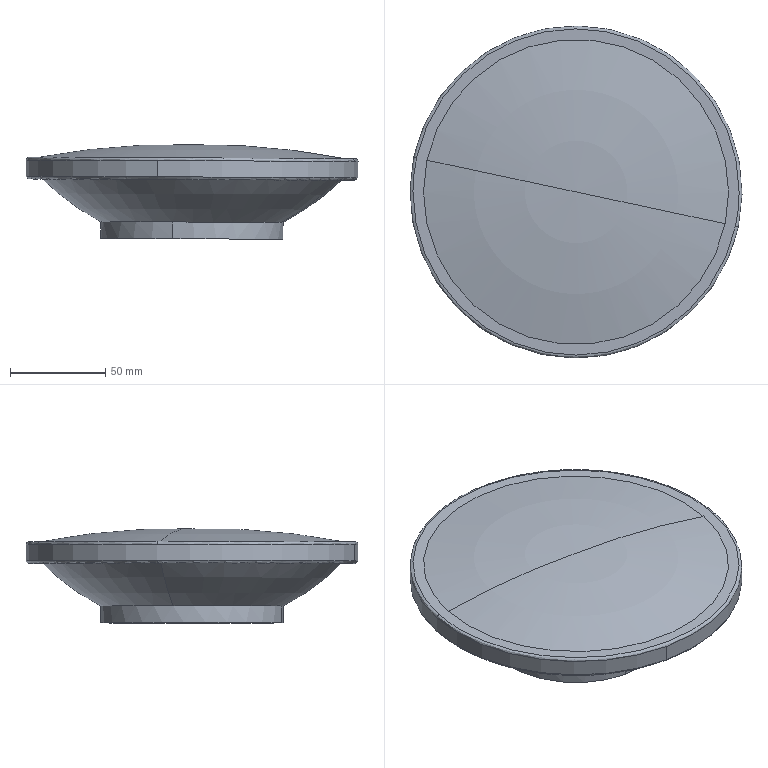Component | SolidWorks | Light-1_GreenLight-1 | 1 solid | 15 faces | box 174.03 x 174 x 49.62 mm | volume 703261 mm3 | cylinder 4 | torus 4 | spline 4 | plane 3 | commonest cylinder face diameters 95.736 x2 174 x2
STEP:
#1=COLOUR_RGB('',0.7922,0.8196,0.9333);
#2=FILL_AREA_STYLE_COLOUR('',#1);
#3=FILL_AREA_STYLE('',(#2));
#4=SURFACE_STYLE_FILL_AREA(#3);
#5=SURFACE_SIDE_STYLE('',(#4));
#6=SURFACE_STYLE_USAGE(.BOTH.,#5);
#7=PRESENTATION_STYLE_ASSIGNMENT((#6));
#8=CARTESIAN_POINT('',(-212.,267.71,12.424));
#9=VERTEX_POINT('',#8);
#10=CARTESIAN_POINT('',(-212.786,264.024,12.427));
#11=VERTEX_POINT('',#10);
#12=CARTESIAN_POINT('',(-212.393,265.867,12.425));
#13=DIRECTION('',(-0.004294,-0.,-1.));
#14=DIRECTION('',(-0.2083,-0.9781,0.0008945));
#15=AXIS2_PLACEMENT_3D('',#12,#13,#14);
#16=CIRCLE('',#15,1.885);
#17=EDGE_CURVE('',#9,#11,#16,.T.);
#18=ORIENTED_EDGE('',*,*,#17,.F.);
#19=CARTESIAN_POINT('',(-211.999,267.71,12.771));
#20=VERTEX_POINT('',#19);
#21=CARTESIAN_POINT('',(-212.,267.71,12.424));
#22=DIRECTION('',(0.004294,0.,1.));
#23=VECTOR('',#22,39.37);
#24=LINE('',#21,#23);
#25=EDGE_CURVE('',#9,#20,#24,.T.);
#26=ORIENTED_EDGE('',*,*,#25,.T.);
#27=CARTESIAN_POINT('',(-210.548,265.474,12.764));
#28=VERTEX_POINT('',#27);
#29=CARTESIAN_POINT('',(-212.392,265.867,12.772));
#30=DIRECTION('',(0.004294,0.,1.));
#31=DIRECTION('',(-0.978,0.2083,0.004199));
#32=AXIS2_PLACEMENT_3D('',#29,#30,#31);
#33=CIRCLE('',#32,1.885);
#34=EDGE_CURVE('',#28,#20,#33,.T.);
#35=ORIENTED_EDGE('',*,*,#34,.F.);
#36=CARTESIAN_POINT('',(-212.784,264.024,12.774));
#37=VERTEX_POINT('',#36);
#38=CARTESIAN_POINT('',(-212.392,265.867,12.772));
#39=DIRECTION('',(0.004294,0.,1.));
#40=DIRECTION('',(-0.978,0.2083,0.004199));
#41=AXIS2_PLACEMENT_3D('',#38,#39,#40);
#42=CIRCLE('',#41,1.885);
#43=EDGE_CURVE('',#37,#28,#42,.T.);
#44=ORIENTED_EDGE('',*,*,#43,.F.);
#45=CARTESIAN_POINT('',(-212.786,264.024,12.427));
#46=DIRECTION('',(0.004294,0.,1.));
#47=VECTOR('',#46,39.37);
#48=LINE('',#45,#47);
#49=EDGE_CURVE('',#11,#37,#48,.T.);
#50=ORIENTED_EDGE('',*,*,#49,.F.);
#51=EDGE_LOOP('',(#18,#26,#35,#44,#50));
#52=FACE_OUTER_BOUND('',#51,.T.);
#53=CARTESIAN_POINT('',(-212.393,265.867,12.425));
#54=DIRECTION('',(0.004294,0.,1.));
#55=DIRECTION('',(-0.2083,-0.9781,0.0008945));
#56=AXIS2_PLACEMENT_3D('',#53,#54,#55);
#57=CYLINDRICAL_SURFACE('',#56,1.885);
#58=ADVANCED_FACE('',(#52),#57,.T.);
#59=CARTESIAN_POINT('',(-214.235,266.26,12.78));
#60=VERTEX_POINT('',#59);
#61=CARTESIAN_POINT('',(-212.392,265.867,12.772));
#62=DIRECTION('',(0.004294,0.,1.));
#63=DIRECTION('',(-0.978,0.2083,0.004199));
#64=AXIS2_PLACEMENT_3D('',#61,#62,#63);
#65=CIRCLE('',#64,1.885);
#66=EDGE_CURVE('',#60,#37,#65,.T.);
#67=ORIENTED_EDGE('',*,*,#66,.T.);
#68=ORIENTED_EDGE('',*,*,#43,.T.);
#69=CARTESIAN_POINT('',(-209.309,265.211,13.689));
#70=VERTEX_POINT('',#69);
#71=CARTESIAN_POINT('',(-212.93,265.986,17.433));
#72=DIRECTION('',(-0.2083,-0.9781,0.0008945));
#73=DIRECTION('',(0.9781,-0.2083,0.));
#74=AXIS2_PLACEMENT_3D('',#71,#72,#73);
#75=CIRCLE('',#74,5.266);
#76=EDGE_CURVE('',#28,#70,#75,.T.);
#77=ORIENTED_EDGE('',*,*,#76,.T.);
#78=CARTESIAN_POINT('',(-215.466,266.523,13.716));
#79=VERTEX_POINT('',#78);
#80=CARTESIAN_POINT('',(-212.388,265.867,13.702));
#81=DIRECTION('',(-0.004294,-0.,-1.));
#82=DIRECTION('',(-0.978,0.2083,0.004199));
#83=AXIS2_PLACEMENT_3D('',#80,#81,#82);
#84=CIRCLE('',#83,3.148);
#85=EDGE_CURVE('',#70,#79,#84,.T.);
#86=ORIENTED_EDGE('',*,*,#85,.T.);
#87=CARTESIAN_POINT('',(-211.813,265.748,17.428));
#88=DIRECTION('',(0.2083,0.9781,-0.0008945));
#89=DIRECTION('',(-0.9781,0.2083,0.));
#90=AXIS2_PLACEMENT_3D('',#87,#88,#89);
#91=CIRCLE('',#90,5.266);
#92=EDGE_CURVE('',#60,#79,#91,.T.);
#93=ORIENTED_EDGE('',*,*,#92,.F.);
#94=EDGE_LOOP('',(#67,#68,#77,#86,#93));
#95=FACE_OUTER_BOUND('',#94,.T.);
#96=CARTESIAN_POINT('',(-212.372,265.867,17.431));
#97=DIRECTION('',(0.004294,0.,1.));
#98=DIRECTION('',(-0.978,0.2083,0.004199));
#99=AXIS2_PLACEMENT_3D('',#96,#97,#98);
#100=TOROIDAL_SURFACE('',#99,-0.5709,5.266);
#101=ADVANCED_FACE('',(#95),#100,.T.);
#102=CARTESIAN_POINT('',(-211.674,269.217,13.699));
#103=VERTEX_POINT('',#102);
#104=CARTESIAN_POINT('',(-209.038,265.154,13.688));
#105=VERTEX_POINT('',#104);
#106=CARTESIAN_POINT('',(-212.388,265.867,13.702));
#107=DIRECTION('',(-0.004294,-0.,-1.));
#108=DIRECTION('',(0.978,-0.2083,-0.004199));
#109=AXIS2_PLACEMENT_3D('',#106,#107,#108);
#110=CIRCLE('',#109,3.425);
#111=EDGE_CURVE('',#103,#105,#110,.T.);
#112=ORIENTED_EDGE('',*,*,#111,.F.);
#113=CARTESIAN_POINT('',(-211.673,269.217,14.034));
#114=VERTEX_POINT('',#113);
#115=CARTESIAN_POINT('',(-211.674,269.217,13.699));
#116=DIRECTION('',(0.004294,0.,1.));
#117=VECTOR('',#116,39.37);
#118=LINE('',#115,#117);
#119=EDGE_CURVE('',#103,#114,#118,.T.);
#120=ORIENTED_EDGE('',*,*,#119,.T.);
#121=CARTESIAN_POINT('',(-209.036,265.154,14.023));
#122=VERTEX_POINT('',#121);
#123=CARTESIAN_POINT('',(-212.386,265.867,14.037));
#124=DIRECTION('',(0.004294,0.,1.));
#125=DIRECTION('',(-0.978,0.2083,0.004199));
#126=AXIS2_PLACEMENT_3D('',#123,#124,#125);
#127=CIRCLE('',#126,3.425);
#128=EDGE_CURVE('',#122,#114,#127,.T.);
#129=ORIENTED_EDGE('',*,*,#128,.F.);
#130=CARTESIAN_POINT('',(-213.1,262.517,14.04));
#131=VERTEX_POINT('',#130);
#132=CARTESIAN_POINT('',(-212.386,265.867,14.037));
#133=DIRECTION('',(0.004294,0.,1.));
#134=DIRECTION('',(-0.978,0.2083,0.004199));
#135=AXIS2_PLACEMENT_3D('',#132,#133,#134);
#136=CIRCLE('',#135,3.425);
#137=EDGE_CURVE('',#131,#122,#136,.T.);
#138=ORIENTED_EDGE('',*,*,#137,.F.);
#139=CARTESIAN_POINT('',(-213.101,262.517,13.705));
#140=VERTEX_POINT('',#139);
#141=CARTESIAN_POINT('',(-213.101,262.517,13.705));
#142=DIRECTION('',(0.004294,0.,1.));
#143=VECTOR('',#142,39.37);
#144=LINE('',#141,#143);
#145=EDGE_CURVE('',#140,#131,#144,.T.);
#146=ORIENTED_EDGE('',*,*,#145,.F.);
#147=CARTESIAN_POINT('',(-212.388,265.867,13.702));
#148=DIRECTION('',(-0.004294,-0.,-1.));
#149=DIRECTION('',(-0.978,0.2083,0.004199));
#150=AXIS2_PLACEMENT_3D('',#147,#148,#149);
#151=CIRCLE('',#150,3.425);
#152=EDGE_CURVE('',#105,#140,#151,.T.);
#153=ORIENTED_EDGE('',*,*,#152,.F.);
#154=EDGE_LOOP('',(#112,#120,#129,#138,#146,#153));
#155=FACE_OUTER_BOUND('',#154,.T.);
#156=CARTESIAN_POINT('',(-212.388,265.867,13.702));
#157=DIRECTION('',(0.004294,0.,1.));
#158=DIRECTION('',(-0.2083,-0.9781,0.0008945));
#159=AXIS2_PLACEMENT_3D('',#156,#157,#158);
#160=CYLINDRICAL_SURFACE('',#159,3.425);
#161=ADVANCED_FACE('',(#155),#160,.T.);
#162=CARTESIAN_POINT('',(-209.307,265.211,14.083));
#163=VERTEX_POINT('',#162);
#164=CARTESIAN_POINT('',(-215.465,266.523,14.109));
#165=VERTEX_POINT('',#164);
#166=CARTESIAN_POINT('',(-212.386,265.867,14.096));
#167=DIRECTION('',(-0.004294,-0.,-1.));
#168=DIRECTION('',(-0.978,0.2083,0.004199));
#169=AXIS2_PLACEMENT_3D('',#166,#167,#168);
#170=CIRCLE('',#169,3.148);
#171=EDGE_CURVE('',#163,#165,#170,.T.);
#172=ORIENTED_EDGE('',*,*,#171,.F.);
#173=CARTESIAN_POINT('',(-212.385,265.867,14.366));
#174=VERTEX_POINT('',#173);
#175=CARTESIAN_POINT('',(-212.167,265.807,-0.7305));
#176=DIRECTION('',(-0.2083,-0.9781,0.0008945));
#177=DIRECTION('',(0.9781,-0.2083,0.));
#178=AXIS2_PLACEMENT_3D('',#175,#176,#177);
#179=CIRCLE('',#178,15.099);
#180=EDGE_CURVE('',#163,#174,#179,.T.);
#181=ORIENTED_EDGE('',*,*,#180,.T.);
#182=CARTESIAN_POINT('',(-212.732,265.927,-0.7281));
#183=DIRECTION('',(0.2083,0.9781,-0.0008945));
#184=DIRECTION('',(-0.9781,0.2083,0.));
#185=AXIS2_PLACEMENT_3D('',#182,#183,#184);
#186=CIRCLE('',#185,15.099);
#187=EDGE_CURVE('',#165,#174,#186,.T.);
#188=ORIENTED_EDGE('',*,*,#187,.F.);
#189=EDGE_LOOP('',(#172,#181,#188));
#190=FACE_OUTER_BOUND('',#189,.T.);
#191=CARTESIAN_POINT('',(-212.45,265.867,-0.7293));
#192=DIRECTION('',(0.004294,0.,1.));
#193=DIRECTION('',(-0.978,0.2083,0.004199));
#194=AXIS2_PLACEMENT_3D('',#191,#192,#193);
#195=TOROIDAL_SURFACE('',#194,0.2891,15.099);
#196=ADVANCED_FACE('',(#190),#195,.T.);
#197=ORIENTED_EDGE('',*,*,#25,.F.);
#198=CARTESIAN_POINT('',(-212.393,265.867,12.425));
#199=DIRECTION('',(-0.004294,-0.,-1.));
#200=DIRECTION('',(-0.2083,-0.9781,0.0008945));
#201=AXIS2_PLACEMENT_3D('',#198,#199,#200);
#202=CIRCLE('',#201,1.885);
#203=EDGE_CURVE('',#11,#9,#202,.T.);
#204=ORIENTED_EDGE('',*,*,#203,.F.);
#205=ORIENTED_EDGE('',*,*,#49,.T.);
#206=ORIENTED_EDGE('',*,*,#66,.F.);
#207=CARTESIAN_POINT('',(-212.392,265.867,12.772));
#208=DIRECTION('',(0.004294,0.,1.));
#209=DIRECTION('',(-0.978,0.2083,0.004199));
#210=AXIS2_PLACEMENT_3D('',#207,#208,#209);
#211=CIRCLE('',#210,1.885);
#212=EDGE_CURVE('',#20,#60,#211,.T.);
#213=ORIENTED_EDGE('',*,*,#212,.F.);
#214=EDGE_LOOP('',(#197,#204,#205,#206,#213));
#215=FACE_OUTER_BOUND('',#214,.T.);
#216=CARTESIAN_POINT('',(-212.393,265.867,12.425));
#217=DIRECTION('',(0.004294,0.,1.));
#218=DIRECTION('',(-0.2083,-0.9781,0.0008945));
#219=AXIS2_PLACEMENT_3D('',#216,#217,#218);
#220=CYLINDRICAL_SURFACE('',#219,1.885);
#221=ADVANCED_FACE('',(#215),#220,.T.);
#222=ORIENTED_EDGE('',*,*,#203,.T.);
#223=ORIENTED_EDGE('',*,*,#17,.T.);
#224=EDGE_LOOP('',(#222,#223));
#225=FACE_OUTER_BOUND('',#224,.T.);
#226=CARTESIAN_POINT('',(-213.861,268.13,12.432));
#227=DIRECTION('',(-0.004294,-0.,-1.));
#228=DIRECTION('',(0.978,-0.2083,-0.004199));
#229=AXIS2_PLACEMENT_3D('',#226,#227,#228);
#230=PLANE('',#229);
#231=ADVANCED_FACE('',(#225),#230,.T.);
#232=ORIENTED_EDGE('',*,*,#76,.F.);
#233=ORIENTED_EDGE('',*,*,#34,.T.);
#234=ORIENTED_EDGE('',*,*,#212,.T.);
#235=ORIENTED_EDGE('',*,*,#92,.T.);
#236=CARTESIAN_POINT('',(-212.388,265.867,13.702));
#237=DIRECTION('',(-0.004294,-0.,-1.));
#238=DIRECTION('',(-0.978,0.2083,0.004199));
#239=AXIS2_PLACEMENT_3D('',#236,#237,#238);
#240=CIRCLE('',#239,3.148);
#241=EDGE_CURVE('',#79,#70,#240,.T.);
#242=ORIENTED_EDGE('',*,*,#241,.T.);
#243=EDGE_LOOP('',(#232,#233,#234,#235,#242));
#244=FACE_OUTER_BOUND('',#243,.T.);
#245=CARTESIAN_POINT('',(-212.372,265.867,17.431));
#246=DIRECTION('',(0.004294,0.,1.));
#247=DIRECTION('',(-0.978,0.2083,0.004199));
#248=AXIS2_PLACEMENT_3D('',#245,#246,#247);
#249=TOROIDAL_SURFACE('',#248,-0.5709,5.266);
#250=ADVANCED_FACE('',(#244),#249,.T.);
#251=ORIENTED_EDGE('',*,*,#241,.F.);
#252=ORIENTED_EDGE('',*,*,#85,.F.);
#253=EDGE_LOOP('',(#251,#252));
#254=FACE_BOUND('',#253,.T.);
#255=CARTESIAN_POINT('',(-209.202,265.189,13.689));
#256=VERTEX_POINT('',#255);
#257=CARTESIAN_POINT('',(-215.573,266.546,13.716));
#258=VERTEX_POINT('',#257);
#259=CARTESIAN_POINT('',(-209.202,265.189,13.689));
#260=CARTESIAN_POINT('',(-210.559,258.817,13.695));
#261=CARTESIAN_POINT('',(-216.93,260.174,13.722));
#262=CARTESIAN_POINT('',(-215.573,266.546,13.716));
#263=(BOUNDED_CURVE()B_SPLINE_CURVE(3,(#259,#260,#261,#262),.UNSPECIFIED.,.F.,.T.)B_SPLINE_CURVE_WITH_KNOTS((4,4),(0.,0.2611),.UNSPECIFIED.)CURVE()GEOMETRIC_REPRESENTATION_ITEM()RATIONAL_B_SPLINE_CURVE((0.9317,0.3106,0.3106,0.9317))REPRESENTATION_ITEM(''));
#264=EDGE_CURVE('',#256,#258,#263,.T.);
#265=ORIENTED_EDGE('',*,*,#264,.T.);
#266=CARTESIAN_POINT('',(-215.573,266.546,13.716));
#267=CARTESIAN_POINT('',(-214.216,272.917,13.71));
#268=CARTESIAN_POINT('',(-207.845,271.56,13.683));
#269=CARTESIAN_POINT('',(-209.202,265.189,13.689));
#270=(BOUNDED_CURVE()B_SPLINE_CURVE(3,(#266,#267,#268,#269),.UNSPECIFIED.,.F.,.T.)B_SPLINE_CURVE_WITH_KNOTS((4,4),(0.,0.2611),.UNSPECIFIED.)CURVE()GEOMETRIC_REPRESENTATION_ITEM()RATIONAL_B_SPLINE_CURVE((0.9317,0.3106,0.3106,0.9317))REPRESENTATION_ITEM(''));
#271=EDGE_CURVE('',#258,#256,#270,.T.);
#272=ORIENTED_EDGE('',*,*,#271,.T.);
#273=EDGE_LOOP('',(#265,#272));
#274=FACE_OUTER_BOUND('',#273,.T.);
#275=CARTESIAN_POINT('',(-214.925,269.778,13.713));
#276=DIRECTION('',(-0.004294,-0.,-1.));
#277=DIRECTION('',(0.978,-0.2083,-0.004199));
#278=AXIS2_PLACEMENT_3D('',#275,#276,#277);
#279=PLANE('',#278);
#280=ADVANCED_FACE('',(#254,#274),#279,.T.);
#281=CARTESIAN_POINT('',(-215.738,266.581,13.717));
#282=VERTEX_POINT('',#281);
#283=CARTESIAN_POINT('',(-215.573,266.546,13.716));
#284=CARTESIAN_POINT('',(-215.609,266.553,13.628));
#285=CARTESIAN_POINT('',(-215.702,266.573,13.628));
#286=CARTESIAN_POINT('',(-215.738,266.581,13.717));
#287=(BOUNDED_CURVE()B_SPLINE_CURVE(3,(#283,#284,#285,#286),.UNSPECIFIED.,.F.,.T.)B_SPLINE_CURVE_WITH_KNOTS((4,4),(0.05033,0.9497),.UNSPECIFIED.)CURVE()GEOMETRIC_REPRESENTATION_ITEM()RATIONAL_B_SPLINE_CURVE((0.9317,0.5462,0.5462,0.9317))REPRESENTATION_ITEM(''));
#288=EDGE_CURVE('',#258,#282,#287,.T.);
#289=ORIENTED_EDGE('',*,*,#288,.T.);
#290=CARTESIAN_POINT('',(-212.388,265.867,13.702));
#291=DIRECTION('',(-0.004294,-0.,-1.));
#292=DIRECTION('',(0.978,-0.2083,-0.004199));
#293=AXIS2_PLACEMENT_3D('',#290,#291,#292);
#294=CIRCLE('',#293,3.425);
#295=EDGE_CURVE('',#282,#103,#294,.T.);
#296=ORIENTED_EDGE('',*,*,#295,.T.);
#297=ORIENTED_EDGE('',*,*,#111,.T.);
#298=CARTESIAN_POINT('',(-209.038,265.154,13.688));
#299=CARTESIAN_POINT('',(-209.073,265.161,13.6));
#300=CARTESIAN_POINT('',(-209.167,265.181,13.6));
#301=CARTESIAN_POINT('',(-209.202,265.189,13.689));
#302=(BOUNDED_CURVE()B_SPLINE_CURVE(3,(#298,#299,#300,#301),.UNSPECIFIED.,.F.,.T.)B_SPLINE_CURVE_WITH_KNOTS((4,4),(0.05033,0.9497),.UNSPECIFIED.)CURVE()GEOMETRIC_REPRESENTATION_ITEM()RATIONAL_B_SPLINE_CURVE((0.9317,0.5462,0.5462,0.9317))REPRESENTATION_ITEM(''));
#303=EDGE_CURVE('',#105,#256,#302,.T.);
#304=ORIENTED_EDGE('',*,*,#303,.T.);
#305=ORIENTED_EDGE('',*,*,#271,.F.);
#306=EDGE_LOOP('',(#289,#296,#297,#304,#305));
#307=FACE_OUTER_BOUND('',#306,.T.);
#308=CARTESIAN_POINT('',(-209.035,265.153,13.697));
#309=CARTESIAN_POINT('',(-207.606,271.859,13.69));
#310=CARTESIAN_POINT('',(-214.312,273.287,13.719));
#311=CARTESIAN_POINT('',(-215.74,266.581,13.725));
#312=CARTESIAN_POINT('',(-209.066,265.159,13.59));
#313=CARTESIAN_POINT('',(-207.651,271.804,13.584));
#314=CARTESIAN_POINT('',(-214.295,273.219,13.613));
#315=CARTESIAN_POINT('',(-215.71,266.575,13.619));
#316=CARTESIAN_POINT('',(-209.174,265.183,13.591));
#317=CARTESIAN_POINT('',(-207.805,271.61,13.585));
#318=CARTESIAN_POINT('',(-214.233,272.979,13.613));
#319=CARTESIAN_POINT('',(-215.602,266.552,13.618));
#320=CARTESIAN_POINT('',(-209.205,265.189,13.697));
#321=CARTESIAN_POINT('',(-207.849,271.554,13.691));
#322=CARTESIAN_POINT('',(-214.214,272.91,13.719));
#323=CARTESIAN_POINT('',(-215.57,266.545,13.725));
#324=(BOUNDED_SURFACE()B_SPLINE_SURFACE(3,3,((#308,#309,#310,#311),(#312,#313,#314,#315),(#316,#317,#318,#319),(#320,#321,#322,#323)),.UNSPECIFIED.,.F.,.F.,.F.)B_SPLINE_SURFACE_WITH_KNOTS((4,4),(4,4),(0.,1.),(0.,1.),.UNSPECIFIED.)GEOMETRIC_REPRESENTATION_ITEM()RATIONAL_B_SPLINE_SURFACE(((1.,0.3333,0.3333,1.),(0.5234,0.1745,0.1745,0.5234),(0.5234,0.1745,0.1745,0.5234),(1.,0.3333,0.3333,1.)))REPRESENTATION_ITEM('')SURFACE());
#325=ADVANCED_FACE('',(#307),#324,.T.);
#326=ORIENTED_EDGE('',*,*,#152,.T.);
#327=CARTESIAN_POINT('',(-212.388,265.867,13.702));
#328=DIRECTION('',(-0.004294,-0.,-1.));
#329=DIRECTION('',(-0.978,0.2083,0.004199));
#330=AXIS2_PLACEMENT_3D('',#327,#328,#329);
#331=CIRCLE('',#330,3.425);
#332=EDGE_CURVE('',#140,#282,#331,.T.);
#333=ORIENTED_EDGE('',*,*,#332,.T.);
#334=ORIENTED_EDGE('',*,*,#288,.F.);
#335=ORIENTED_EDGE('',*,*,#264,.F.);
#336=ORIENTED_EDGE('',*,*,#303,.F.);
#337=EDGE_LOOP('',(#326,#333,#334,#335,#336));
#338=FACE_OUTER_BOUND('',#337,.T.);
#339=CARTESIAN_POINT('',(-215.74,266.581,13.725));
#340=CARTESIAN_POINT('',(-217.169,259.875,13.732));
#341=CARTESIAN_POINT('',(-210.463,258.447,13.703));
#342=CARTESIAN_POINT('',(-209.035,265.153,13.697));
#343=CARTESIAN_POINT('',(-215.71,266.575,13.619));
#344=CARTESIAN_POINT('',(-217.125,259.931,13.625));
#345=CARTESIAN_POINT('',(-210.481,258.515,13.596));
#346=CARTESIAN_POINT('',(-209.066,265.159,13.59));
#347=CARTESIAN_POINT('',(-215.602,266.552,13.618));
#348=CARTESIAN_POINT('',(-216.971,260.124,13.624));
#349=CARTESIAN_POINT('',(-210.543,258.755,13.597));
#350=CARTESIAN_POINT('',(-209.174,265.183,13.591));
#351=CARTESIAN_POINT('',(-215.57,266.545,13.725));
#352=CARTESIAN_POINT('',(-216.926,260.18,13.73));
#353=CARTESIAN_POINT('',(-210.561,258.824,13.703));
#354=CARTESIAN_POINT('',(-209.205,265.189,13.697));
#355=(BOUNDED_SURFACE()B_SPLINE_SURFACE(3,3,((#339,#340,#341,#342),(#343,#344,#345,#346),(#347,#348,#349,#350),(#351,#352,#353,#354)),.UNSPECIFIED.,.F.,.F.,.F.)B_SPLINE_SURFACE_WITH_KNOTS((4,4),(4,4),(0.,1.),(0.,1.),.UNSPECIFIED.)GEOMETRIC_REPRESENTATION_ITEM()RATIONAL_B_SPLINE_SURFACE(((1.,0.3333,0.3333,1.),(0.5234,0.1745,0.1745,0.5234),(0.5234,0.1745,0.1745,0.5234),(1.,0.3333,0.3333,1.)))REPRESENTATION_ITEM('')SURFACE());
#356=ADVANCED_FACE('',(#338),#355,.T.);
#357=ORIENTED_EDGE('',*,*,#119,.F.);
#358=ORIENTED_EDGE('',*,*,#295,.F.);
#359=ORIENTED_EDGE('',*,*,#332,.F.);
#360=ORIENTED_EDGE('',*,*,#145,.T.);
#361=CARTESIAN_POINT('',(-215.736,266.581,14.051));
#362=VERTEX_POINT('',#361);
#363=CARTESIAN_POINT('',(-212.386,265.867,14.037));
#364=DIRECTION('',(0.004294,0.,1.));
#365=DIRECTION('',(-0.978,0.2083,0.004199));
#366=AXIS2_PLACEMENT_3D('',#363,#364,#365);
#367=CIRCLE('',#366,3.425);
#368=EDGE_CURVE('',#362,#131,#367,.T.);
#369=ORIENTED_EDGE('',*,*,#368,.F.);
#370=CARTESIAN_POINT('',(-212.386,265.867,14.037));
#371=DIRECTION('',(0.004294,0.,1.));
#372=DIRECTION('',(-0.978,0.2083,0.004199));
#373=AXIS2_PLACEMENT_3D('',#370,#371,#372);
#374=CIRCLE('',#373,3.425);
#375=EDGE_CURVE('',#114,#362,#374,.T.);
#376=ORIENTED_EDGE('',*,*,#375,.F.);
#377=EDGE_LOOP('',(#357,#358,#359,#360,#369,#376));
#378=FACE_OUTER_BOUND('',#377,.T.);
#379=CARTESIAN_POINT('',(-212.388,265.867,13.702));
#380=DIRECTION('',(0.004294,0.,1.));
#381=DIRECTION('',(-0.2083,-0.9781,0.0008945));
#382=AXIS2_PLACEMENT_3D('',#379,#380,#381);
#383=CYLINDRICAL_SURFACE('',#382,3.425);
#384=ADVANCED_FACE('',(#378),#383,.T.);
#385=CARTESIAN_POINT('',(-215.678,266.568,14.11));
#386=VERTEX_POINT('',#385);
#387=CARTESIAN_POINT('',(-215.736,266.581,14.051));
#388=CARTESIAN_POINT('',(-215.736,266.581,14.086));
#389=CARTESIAN_POINT('',(-215.712,266.576,14.11));
#390=CARTESIAN_POINT('',(-215.678,266.568,14.11));
#391=(BOUNDED_CURVE()B_SPLINE_CURVE(3,(#387,#388,#389,#390),.UNSPECIFIED.,.F.,.T.)B_SPLINE_CURVE_WITH_KNOTS((4,4),(0.06314,0.9369),.UNSPECIFIED.)CURVE()GEOMETRIC_REPRESENTATION_ITEM()RATIONAL_B_SPLINE_CURVE((0.9566,0.7698,0.7698,0.9566))REPRESENTATION_ITEM(''));
#392=EDGE_CURVE('',#362,#386,#391,.T.);
#393=ORIENTED_EDGE('',*,*,#392,.T.);
#394=CARTESIAN_POINT('',(-209.094,265.166,14.082));
#395=VERTEX_POINT('',#394);
#396=CARTESIAN_POINT('',(-215.678,266.568,14.11));
#397=CARTESIAN_POINT('',(-214.276,273.153,14.104));
#398=CARTESIAN_POINT('',(-207.691,271.75,14.076));
#399=CARTESIAN_POINT('',(-209.094,265.166,14.082));
#400=(BOUNDED_CURVE()B_SPLINE_CURVE(3,(#396,#397,#398,#399),.UNSPECIFIED.,.F.,.T.)B_SPLINE_CURVE_WITH_KNOTS((4,4),(0.,1.),.UNSPECIFIED.)CURVE()GEOMETRIC_REPRESENTATION_ITEM()RATIONAL_B_SPLINE_CURVE((0.9566,0.3189,0.3189,0.9566))REPRESENTATION_ITEM(''));
#401=EDGE_CURVE('',#386,#395,#400,.T.);
#402=ORIENTED_EDGE('',*,*,#401,.T.);
#403=CARTESIAN_POINT('',(-209.094,265.166,14.082));
#404=CARTESIAN_POINT('',(-209.06,265.159,14.082));
#405=CARTESIAN_POINT('',(-209.036,265.154,14.057));
#406=CARTESIAN_POINT('',(-209.036,265.154,14.023));
#407=(BOUNDED_CURVE()B_SPLINE_CURVE(3,(#403,#404,#405,#406),.UNSPECIFIED.,.F.,.T.)B_SPLINE_CURVE_WITH_KNOTS((4,4),(0.06314,0.9369),.UNSPECIFIED.)CURVE()GEOMETRIC_REPRESENTATION_ITEM()RATIONAL_B_SPLINE_CURVE((0.9566,0.7698,0.7698,0.9566))REPRESENTATION_ITEM(''));
#408=EDGE_CURVE('',#395,#122,#407,.T.);
#409=ORIENTED_EDGE('',*,*,#408,.T.);
#410=ORIENTED_EDGE('',*,*,#128,.T.);
#411=ORIENTED_EDGE('',*,*,#375,.T.);
#412=EDGE_LOOP('',(#393,#402,#409,#410,#411));
#413=FACE_OUTER_BOUND('',#412,.T.);
#414=CARTESIAN_POINT('',(-209.099,265.167,14.082));
#415=CARTESIAN_POINT('',(-207.699,271.74,14.076));
#416=CARTESIAN_POINT('',(-214.272,273.14,14.104));
#417=CARTESIAN_POINT('',(-215.672,266.567,14.11));
#418=CARTESIAN_POINT('',(-209.06,265.159,14.086));
#419=CARTESIAN_POINT('',(-207.643,271.81,14.079));
#420=CARTESIAN_POINT('',(-214.295,273.227,14.108));
#421=CARTESIAN_POINT('',(-215.712,266.576,14.114));
#422=CARTESIAN_POINT('',(-209.032,265.153,14.057));
#423=CARTESIAN_POINT('',(-207.604,271.86,14.051));
#424=CARTESIAN_POINT('',(-214.311,273.289,14.08));
#425=CARTESIAN_POINT('',(-215.74,266.581,14.086));
#426=CARTESIAN_POINT('',(-209.036,265.154,14.017));
#427=CARTESIAN_POINT('',(-207.609,271.853,14.011));
#428=CARTESIAN_POINT('',(-214.309,273.28,14.039));
#429=CARTESIAN_POINT('',(-215.736,266.581,14.046));
#430=(BOUNDED_SURFACE()B_SPLINE_SURFACE(3,3,((#414,#415,#416,#417),(#418,#419,#420,#421),(#422,#423,#424,#425),(#426,#427,#428,#429)),.UNSPECIFIED.,.F.,.F.,.F.)B_SPLINE_SURFACE_WITH_KNOTS((4,4),(4,4),(0.,1.),(0.,1.),.UNSPECIFIED.)GEOMETRIC_REPRESENTATION_ITEM()RATIONAL_B_SPLINE_SURFACE(((1.,0.3333,0.3333,1.),(0.7553,0.2518,0.2518,0.7553),(0.7553,0.2518,0.2518,0.7553),(1.,0.3333,0.3333,1.)))REPRESENTATION_ITEM('')SURFACE());
#431=ADVANCED_FACE('',(#413),#430,.T.);
#432=CARTESIAN_POINT('',(-209.094,265.166,14.082));
#433=CARTESIAN_POINT('',(-210.496,258.581,14.088));
#434=CARTESIAN_POINT('',(-217.081,259.984,14.116));
#435=CARTESIAN_POINT('',(-215.678,266.568,14.11));
#436=(BOUNDED_CURVE()B_SPLINE_CURVE(3,(#432,#433,#434,#435),.UNSPECIFIED.,.F.,.T.)B_SPLINE_CURVE_WITH_KNOTS((4,4),(0.,1.),.UNSPECIFIED.)CURVE()GEOMETRIC_REPRESENTATION_ITEM()RATIONAL_B_SPLINE_CURVE((0.9566,0.3189,0.3189,0.9566))REPRESENTATION_ITEM(''));
#437=EDGE_CURVE('',#395,#386,#436,.T.);
#438=ORIENTED_EDGE('',*,*,#437,.T.);
#439=ORIENTED_EDGE('',*,*,#392,.F.);
#440=ORIENTED_EDGE('',*,*,#368,.T.);
#441=ORIENTED_EDGE('',*,*,#137,.T.);
#442=ORIENTED_EDGE('',*,*,#408,.F.);
#443=EDGE_LOOP('',(#438,#439,#440,#441,#442));
#444=FACE_OUTER_BOUND('',#443,.T.);
#445=CARTESIAN_POINT('',(-215.672,266.567,14.11));
#446=CARTESIAN_POINT('',(-217.072,259.994,14.116));
#447=CARTESIAN_POINT('',(-210.499,258.594,14.088));
#448=CARTESIAN_POINT('',(-209.099,265.167,14.082));
#449=CARTESIAN_POINT('',(-215.712,266.576,14.114));
#450=CARTESIAN_POINT('',(-217.128,259.924,14.12));
#451=CARTESIAN_POINT('',(-210.477,258.507,14.092));
#452=CARTESIAN_POINT('',(-209.06,265.159,14.086));
#453=CARTESIAN_POINT('',(-215.74,266.581,14.086));
#454=CARTESIAN_POINT('',(-217.168,259.874,14.092));
#455=CARTESIAN_POINT('',(-210.461,258.445,14.063));
#456=CARTESIAN_POINT('',(-209.032,265.153,14.057));
#457=CARTESIAN_POINT('',(-215.736,266.581,14.046));
#458=CARTESIAN_POINT('',(-217.163,259.881,14.052));
#459=CARTESIAN_POINT('',(-210.463,258.454,14.023));
#460=CARTESIAN_POINT('',(-209.036,265.154,14.017));
#461=(BOUNDED_SURFACE()B_SPLINE_SURFACE(3,3,((#445,#446,#447,#448),(#449,#450,#451,#452),(#453,#454,#455,#456),(#457,#458,#459,#460)),.UNSPECIFIED.,.F.,.F.,.F.)B_SPLINE_SURFACE_WITH_KNOTS((4,4),(4,4),(0.,1.),(0.,1.),.UNSPECIFIED.)GEOMETRIC_REPRESENTATION_ITEM()RATIONAL_B_SPLINE_SURFACE(((1.,0.3333,0.3333,1.),(0.7553,0.2518,0.2518,0.7553),(0.7553,0.2518,0.2518,0.7553),(1.,0.3333,0.3333,1.)))REPRESENTATION_ITEM('')SURFACE());
#462=ADVANCED_FACE('',(#444),#461,.T.);
#463=CARTESIAN_POINT('',(-212.386,265.867,14.096));
#464=DIRECTION('',(-0.004294,-0.,-1.));
#465=DIRECTION('',(-0.978,0.2083,0.004199));
#466=AXIS2_PLACEMENT_3D('',#463,#464,#465);
#467=CIRCLE('',#466,3.148);
#468=EDGE_CURVE('',#165,#163,#467,.T.);
#469=ORIENTED_EDGE('',*,*,#468,.T.);
#470=ORIENTED_EDGE('',*,*,#171,.T.);
#471=EDGE_LOOP('',(#469,#470));
#472=FACE_BOUND('',#471,.T.);
#473=ORIENTED_EDGE('',*,*,#437,.F.);
#474=ORIENTED_EDGE('',*,*,#401,.F.);
#475=EDGE_LOOP('',(#473,#474));
#476=FACE_OUTER_BOUND('',#475,.T.);
#477=CARTESIAN_POINT('',(-208.344,268.489,14.079));
#478=DIRECTION('',(0.004294,0.,1.));
#479=DIRECTION('',(-0.978,0.2083,0.004199));
#480=AXIS2_PLACEMENT_3D('',#477,#478,#479);
#481=PLANE('',#480);
#482=ADVANCED_FACE('',(#472,#476),#481,.T.);
#483=ORIENTED_EDGE('',*,*,#180,.F.);
#484=ORIENTED_EDGE('',*,*,#468,.F.);
#485=ORIENTED_EDGE('',*,*,#187,.T.);
#486=EDGE_LOOP('',(#483,#484,#485));
#487=FACE_OUTER_BOUND('',#486,.T.);
#488=CARTESIAN_POINT('',(-212.45,265.867,-0.7293));
#489=DIRECTION('',(0.004294,0.,1.));
#490=DIRECTION('',(-0.978,0.2083,0.004199));
#491=AXIS2_PLACEMENT_3D('',#488,#489,#490);
#492=TOROIDAL_SURFACE('',#491,0.2891,15.099);
#493=ADVANCED_FACE('',(#487),#492,.T.);
#494=CLOSED_SHELL('',(#58,#101,#161,#196,#221,#231,#250,#280,#325,#356,#384,#431,#462,#482,#493));
#495=MANIFOLD_SOLID_BREP('',#494);
#496=STYLED_ITEM('',(#7),#495);
#497=PRESENTATION_LAYER_ASSIGNMENT('','',(#496));
#498=CARTESIAN_POINT('',(0.,0.,0.));
#499=DIRECTION('',(0.,0.,1.));
#500=DIRECTION('',(1.,0.,0.));
#501=AXIS2_PLACEMENT_3D('',#498,#499,#500);
#502=(LENGTH_UNIT()NAMED_UNIT(*)SI_UNIT($,.METRE.));
#503=LENGTH_MEASURE_WITH_UNIT(LENGTH_MEASURE(0.0254),#502);
#504=DIMENSIONAL_EXPONENTS(1.,0.,0.,0.,0.,0.,0.);
#505=(CONVERSION_BASED_UNIT('',#503)LENGTH_UNIT()NAMED_UNIT(#504));
#506=UNCERTAINTY_MEASURE_WITH_UNIT(LENGTH_MEASURE(0.00001),#505,'','');
#507=(NAMED_UNIT(*)PLANE_ANGLE_UNIT()SI_UNIT($,.RADIAN.));
#508=(NAMED_UNIT(*)SI_UNIT($,.STERADIAN.)SOLID_ANGLE_UNIT());
#509=(GEOMETRIC_REPRESENTATION_CONTEXT(3)GLOBAL_UNCERTAINTY_ASSIGNED_CONTEXT((#506))GLOBAL_UNIT_ASSIGNED_CONTEXT((#505,#507,#508))REPRESENTATION_CONTEXT('',''));
#510=ADVANCED_BREP_SHAPE_REPRESENTATION('',(#495,#501),#509);
#511=(LENGTH_UNIT()NAMED_UNIT(*)SI_UNIT($,.METRE.));
#512=LENGTH_MEASURE_WITH_UNIT(LENGTH_MEASURE(0.0254),#511);
#513=DIMENSIONAL_EXPONENTS(1.,0.,0.,0.,0.,0.,0.);
#514=(CONVERSION_BASED_UNIT('',#512)LENGTH_UNIT()NAMED_UNIT(#513));
#515=UNCERTAINTY_MEASURE_WITH_UNIT(LENGTH_MEASURE(0.00001),#514,'','');
#516=(NAMED_UNIT(*)PLANE_ANGLE_UNIT()SI_UNIT($,.RADIAN.));
#517=(NAMED_UNIT(*)SI_UNIT($,.STERADIAN.)SOLID_ANGLE_UNIT());
#518=(GEOMETRIC_REPRESENTATION_CONTEXT(3)GLOBAL_UNCERTAINTY_ASSIGNED_CONTEXT((#515))GLOBAL_UNIT_ASSIGNED_CONTEXT((#514,#516,#517))REPRESENTATION_CONTEXT('',''));
#519=MECHANICAL_DESIGN_GEOMETRIC_PRESENTATION_REPRESENTATION('',(#496),#518);